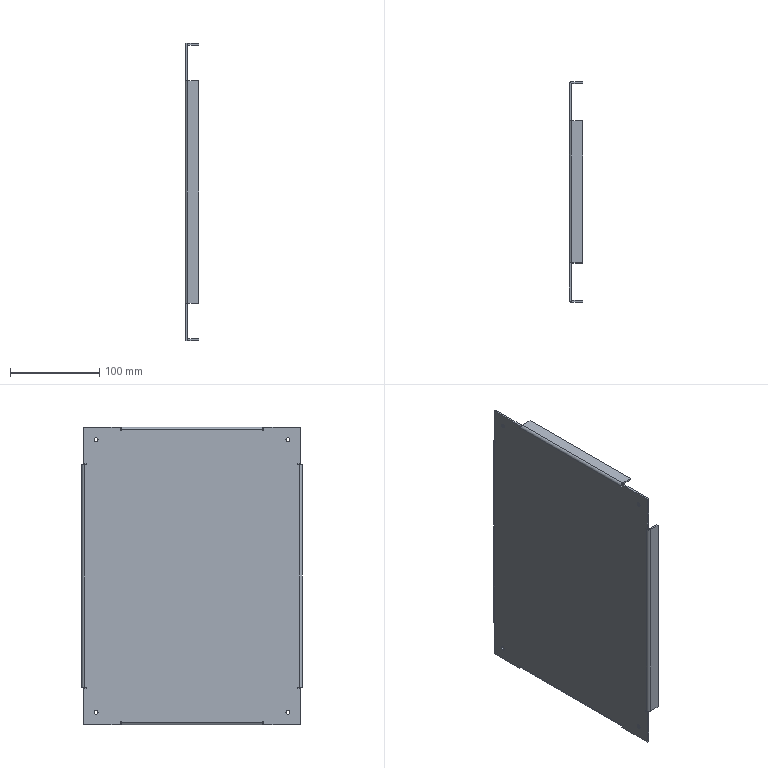Component | SolidWorks | AX00-100.1.1-1_24.1.1-1 | 1 solid | 78 faces | volume 183648 mm3 | plane 62 | cylinder 16 | commonest cylinder face diameters 4.5 x8 5.473 x4 1.473 x4